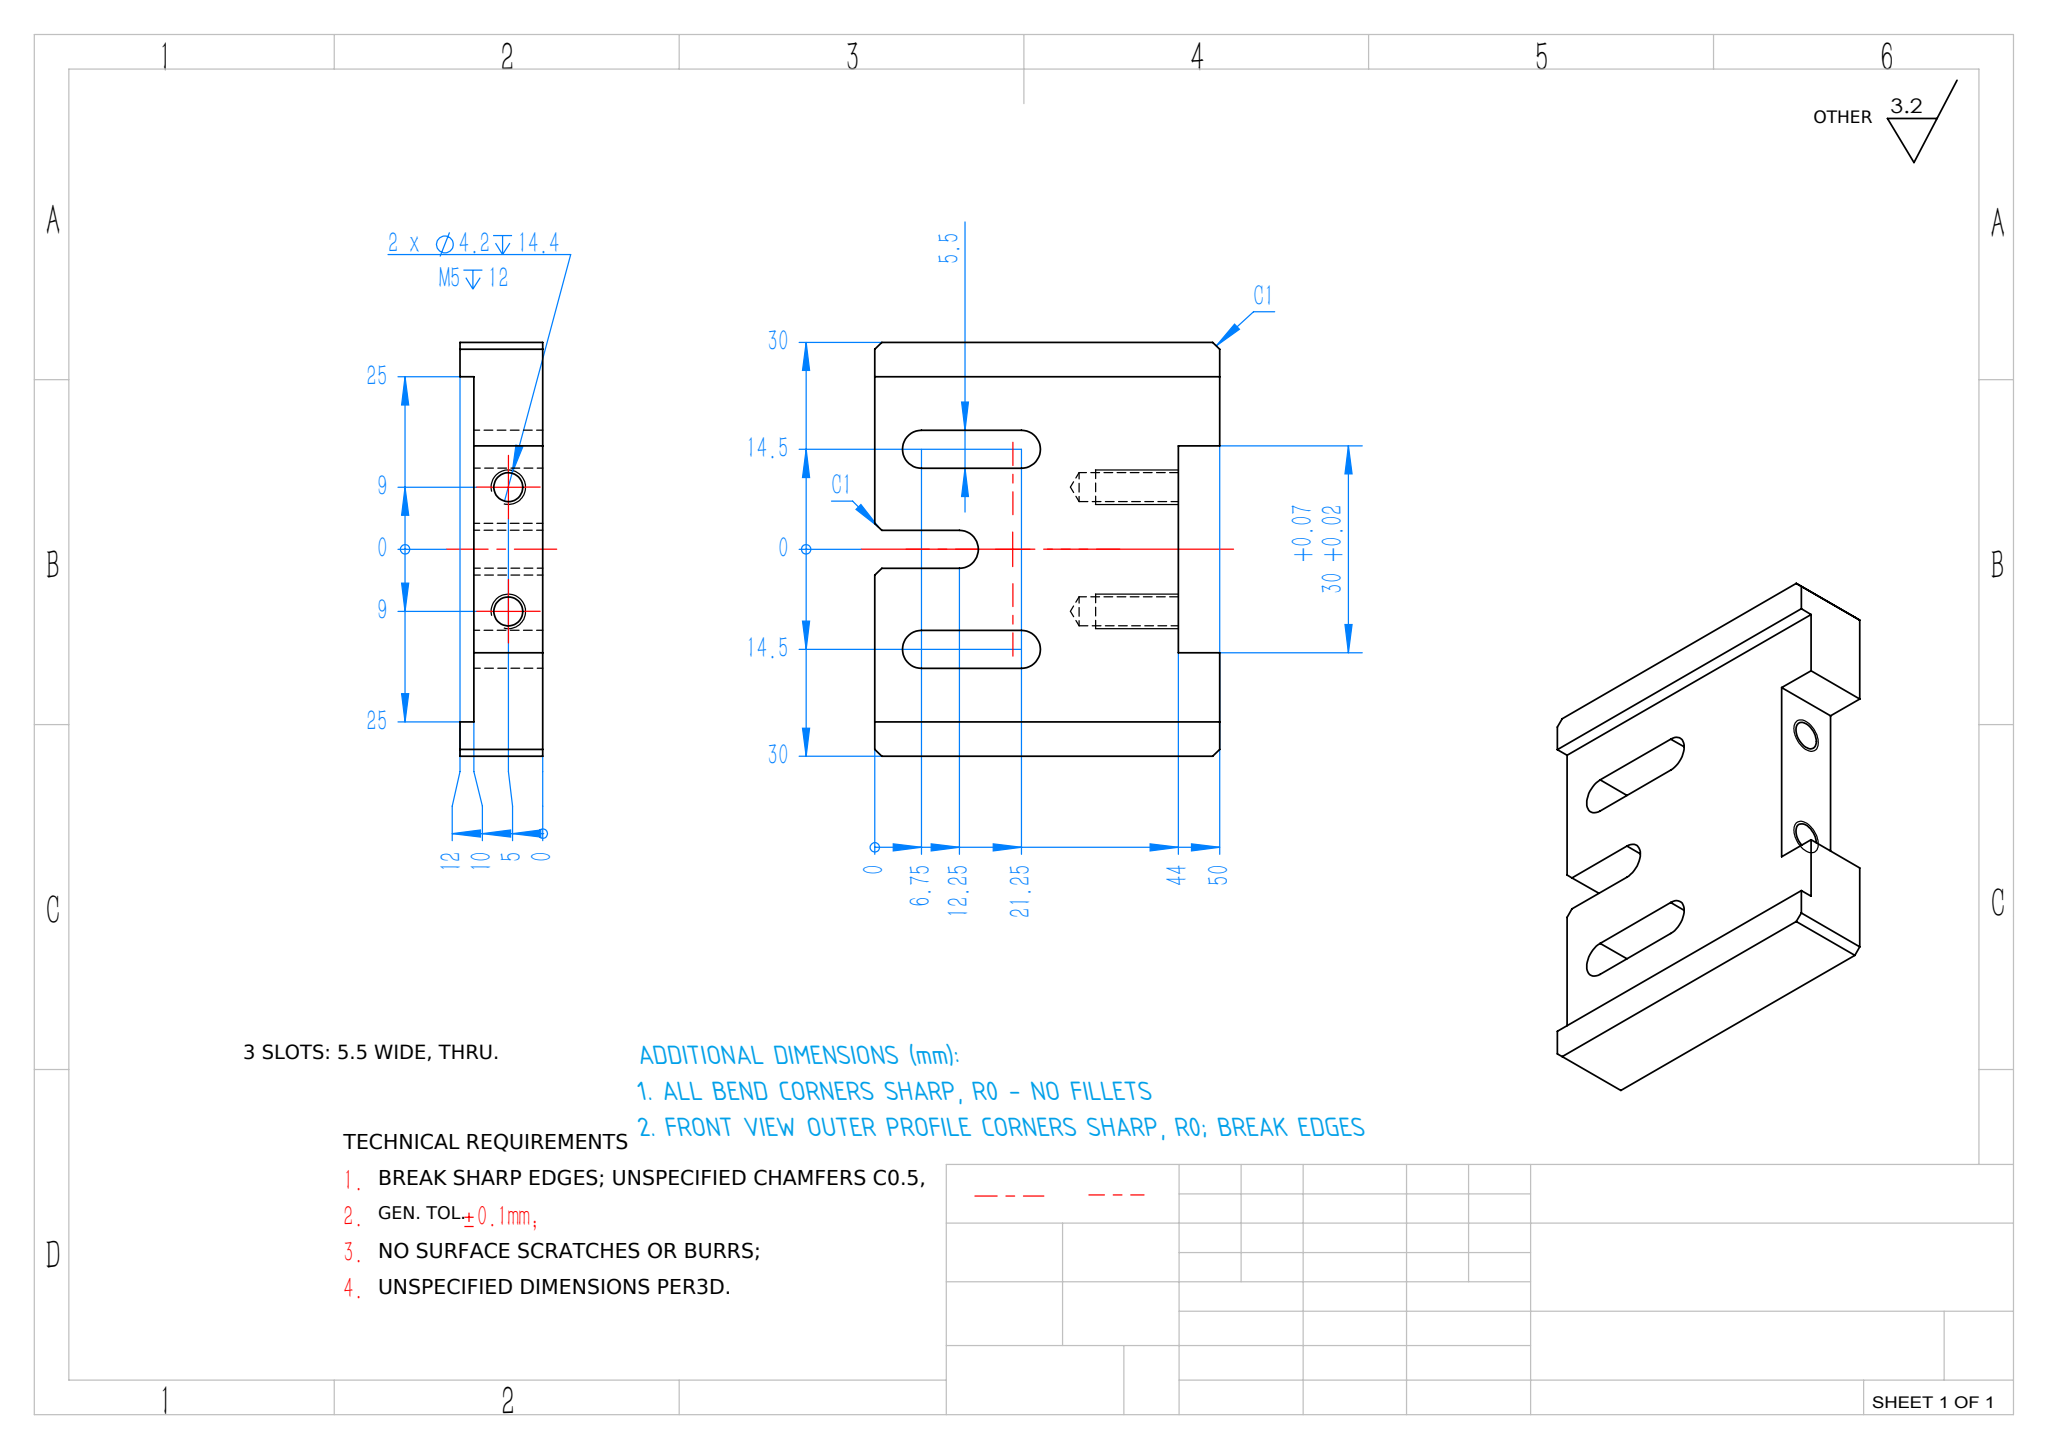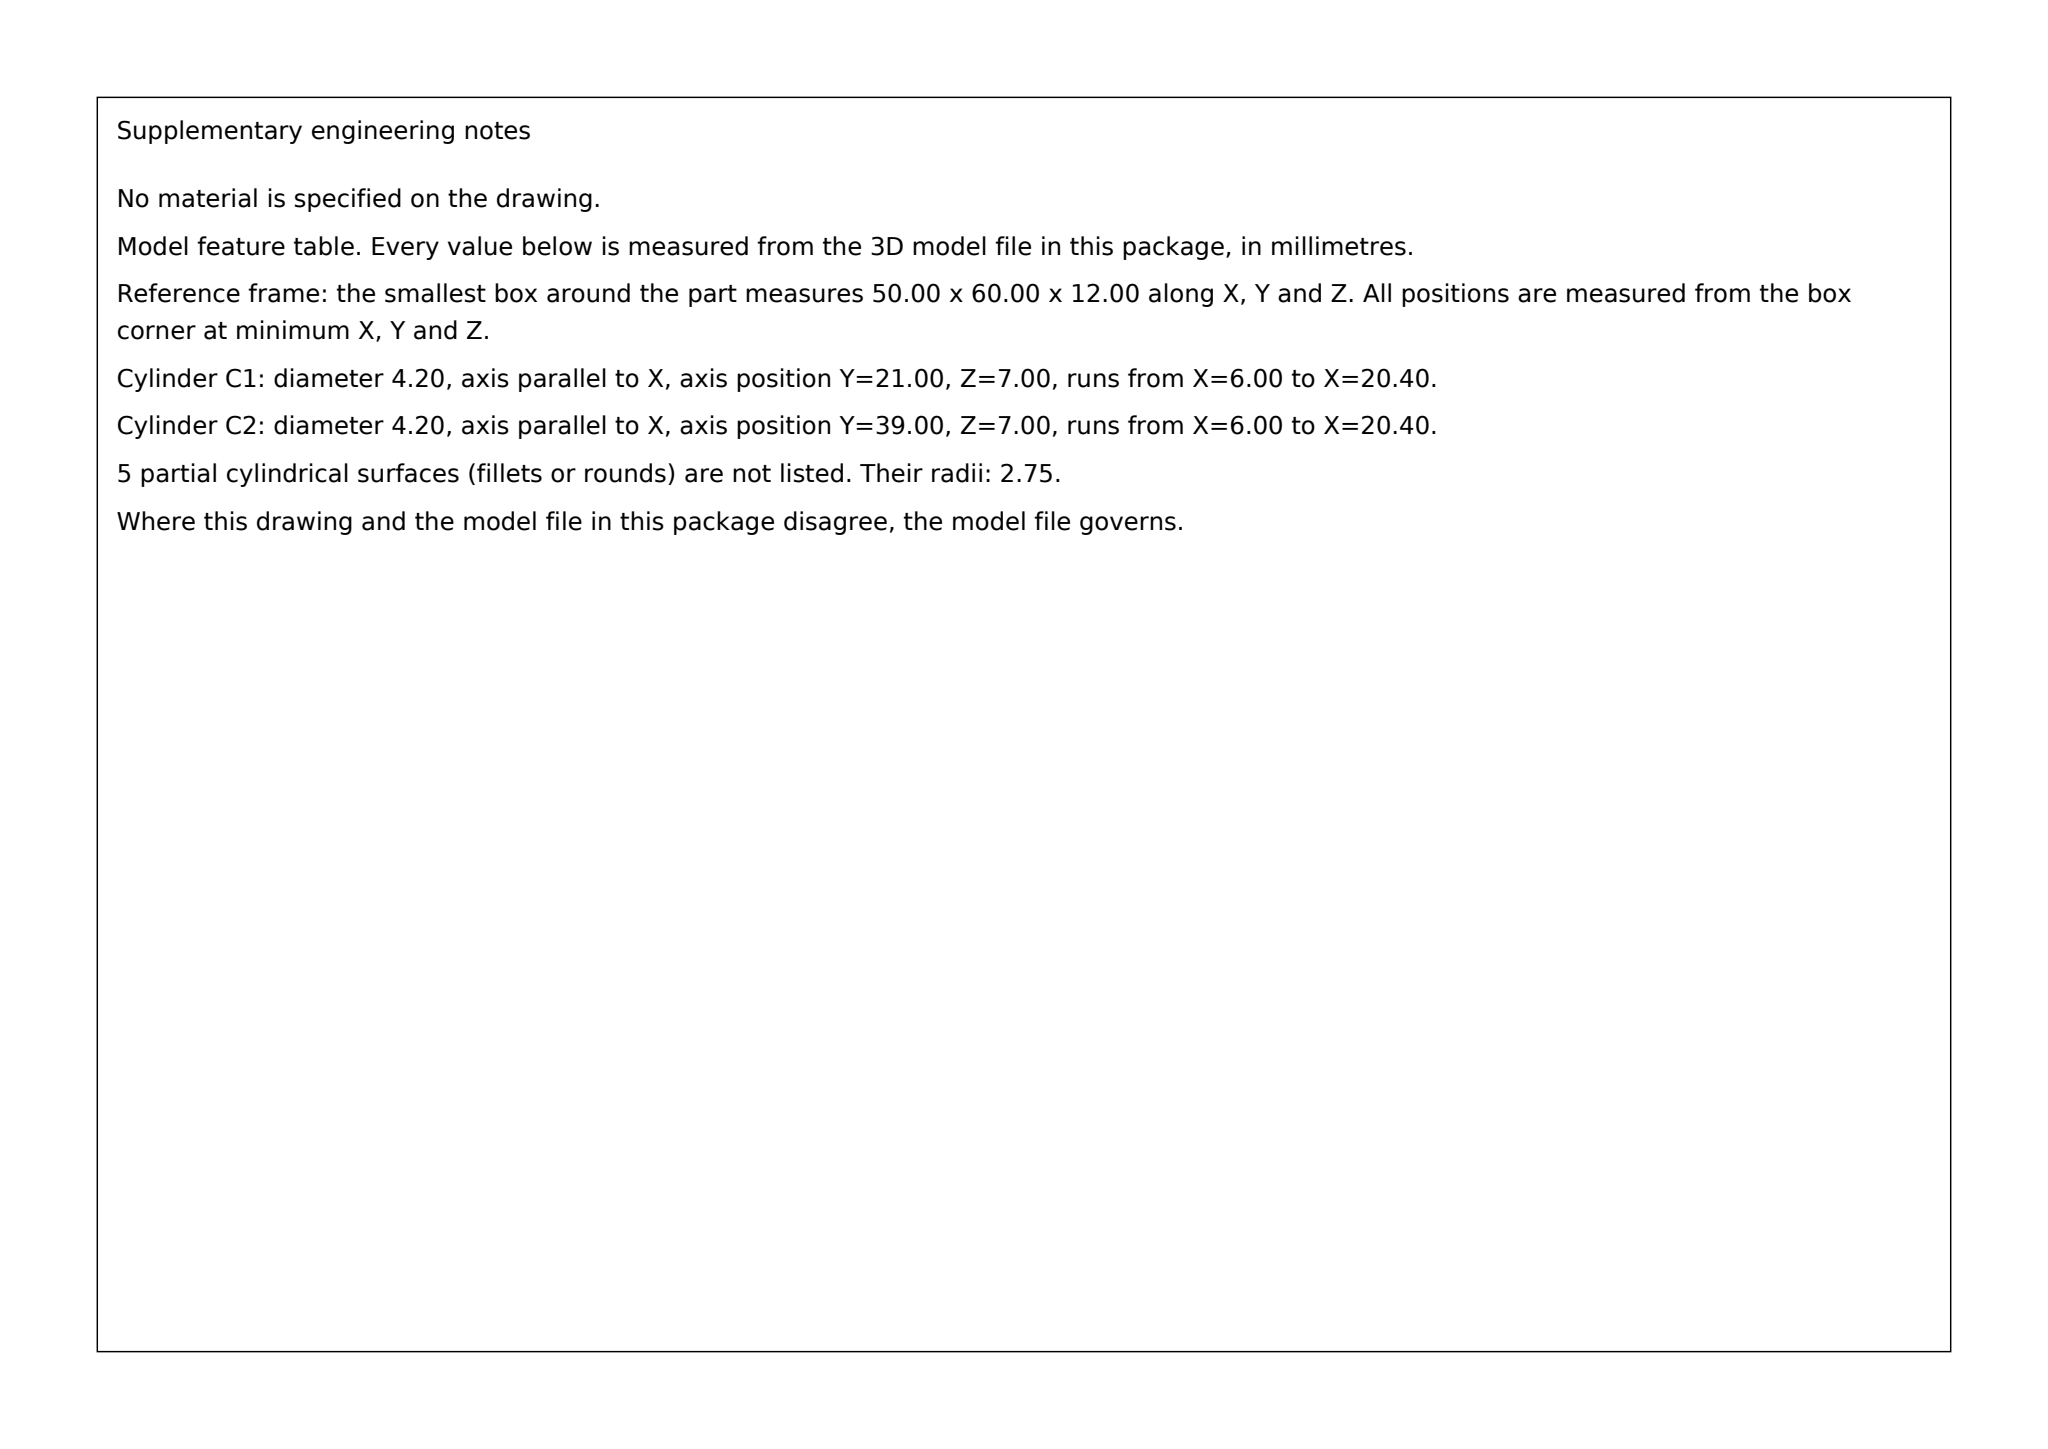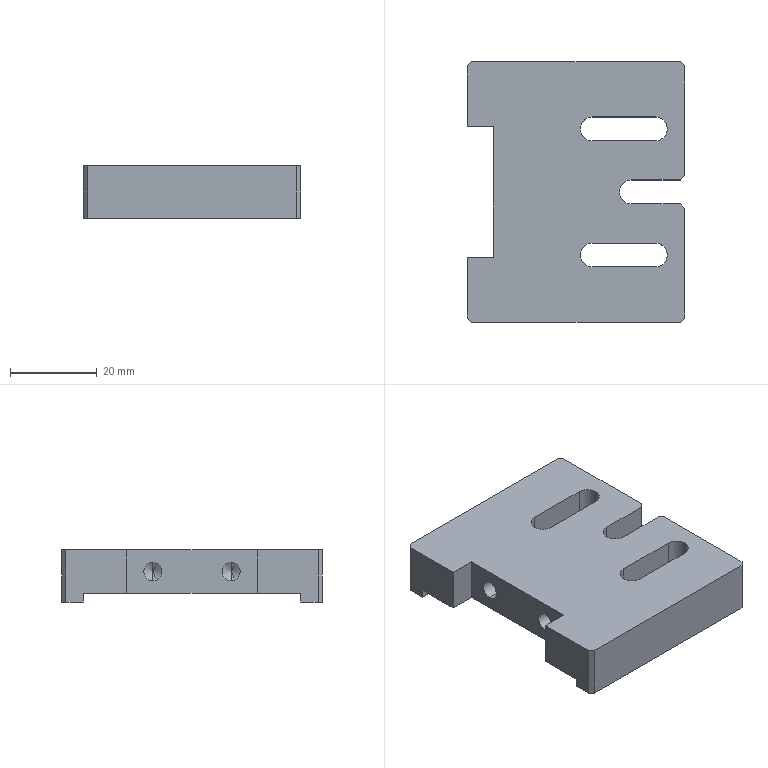Part | SolidWorks | mm | 1 solid | 42 faces | box 50 x 60 x 12 mm | volume 25893 mm3 | plane 27 | cylinder 11 | cone 4 | commonest cylinder face diameters 5.5 x7 4.2 x4